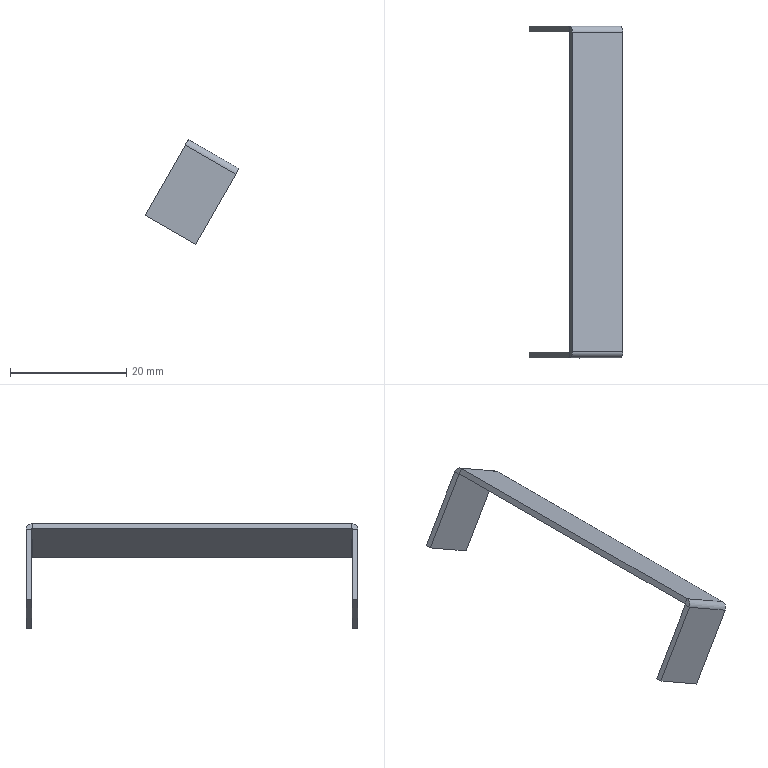Component | SolidWorks | FrontDoorFlangeWelding-2_WireRack-1 | 1 solid | 22 faces | box 16.13 x 57 x 17.99 mm | volume 845 mm3 | plane 18 | cylinder 4 | commonest cylinder face diameters 2.2 x2 0.2 x2
STEP:
#1=CARTESIAN_POINT('',(-0.3547,19.692,56.021));
#2=VERTEX_POINT('',#1);
#3=CARTESIAN_POINT('',(-0.01307,19.692,55.825));
#4=VERTEX_POINT('',#3);
#5=CARTESIAN_POINT('',(-0.3547,19.692,56.021));
#6=DIRECTION('',(0.8677,0.,-0.4971));
#7=VECTOR('',#6,39.37);
#8=LINE('',#5,#7);
#9=EDGE_CURVE('',#2,#4,#8,.T.);
#10=ORIENTED_EDGE('',*,*,#9,.F.);
#11=CARTESIAN_POINT('',(-0.3547,21.849,56.021));
#12=VERTEX_POINT('',#11);
#13=CARTESIAN_POINT('',(-0.3547,21.893,56.021));
#14=DIRECTION('',(0.,-1.,-0.));
#15=VECTOR('',#14,39.37);
#16=LINE('',#13,#15);
#17=EDGE_CURVE('',#12,#2,#16,.T.);
#18=ORIENTED_EDGE('',*,*,#17,.F.);
#19=CARTESIAN_POINT('',(-0.01307,21.849,55.825));
#20=VERTEX_POINT('',#19);
#21=CARTESIAN_POINT('',(-0.01307,21.849,55.825));
#22=DIRECTION('',(-0.8677,-0.,0.4971));
#23=VECTOR('',#22,39.37);
#24=LINE('',#21,#23);
#25=EDGE_CURVE('',#20,#12,#24,.T.);
#26=ORIENTED_EDGE('',*,*,#25,.F.);
#27=CARTESIAN_POINT('',(-0.01307,21.893,55.825));
#28=DIRECTION('',(-0.,1.,0.));
#29=VECTOR('',#28,39.37);
#30=LINE('',#27,#29);
#31=EDGE_CURVE('',#4,#20,#30,.T.);
#32=ORIENTED_EDGE('',*,*,#31,.F.);
#33=EDGE_LOOP('',(#10,#18,#26,#32));
#34=FACE_OUTER_BOUND('',#33,.T.);
#35=CARTESIAN_POINT('',(0.2035,19.647,55.701));
#36=DIRECTION('',(0.4971,-0.,0.8677));
#37=DIRECTION('',(0.8677,0.,-0.4971));
#38=AXIS2_PLACEMENT_3D('',#35,#36,#37);
#39=PLANE('',#38);
#40=ADVANCED_FACE('',(#34),#39,.F.);
#41=CARTESIAN_POINT('',(-0.3351,21.849,56.055));
#42=VERTEX_POINT('',#41);
#43=CARTESIAN_POINT('',(-0.3351,19.692,56.055));
#44=VERTEX_POINT('',#43);
#45=CARTESIAN_POINT('',(-0.3351,21.893,56.055));
#46=DIRECTION('',(0.,-1.,-0.));
#47=VECTOR('',#46,39.37);
#48=LINE('',#45,#47);
#49=EDGE_CURVE('',#42,#44,#48,.T.);
#50=ORIENTED_EDGE('',*,*,#49,.T.);
#51=CARTESIAN_POINT('',(0.006502,19.692,55.859));
#52=VERTEX_POINT('',#51);
#53=CARTESIAN_POINT('',(-0.3351,19.692,56.055));
#54=DIRECTION('',(0.8677,0.,-0.4971));
#55=VECTOR('',#54,39.37);
#56=LINE('',#53,#55);
#57=EDGE_CURVE('',#44,#52,#56,.T.);
#58=ORIENTED_EDGE('',*,*,#57,.T.);
#59=CARTESIAN_POINT('',(0.006502,21.849,55.859));
#60=VERTEX_POINT('',#59);
#61=CARTESIAN_POINT('',(0.006502,21.893,55.859));
#62=DIRECTION('',(-0.,1.,0.));
#63=VECTOR('',#62,39.37);
#64=LINE('',#61,#63);
#65=EDGE_CURVE('',#52,#60,#64,.T.);
#66=ORIENTED_EDGE('',*,*,#65,.T.);
#67=CARTESIAN_POINT('',(0.006502,21.849,55.859));
#68=DIRECTION('',(-0.8677,-0.,0.4971));
#69=VECTOR('',#68,39.37);
#70=LINE('',#67,#69);
#71=EDGE_CURVE('',#60,#42,#70,.T.);
#72=ORIENTED_EDGE('',*,*,#71,.T.);
#73=EDGE_LOOP('',(#50,#58,#66,#72));
#74=FACE_OUTER_BOUND('',#73,.T.);
#75=CARTESIAN_POINT('',(0.2231,19.647,55.735));
#76=DIRECTION('',(0.4971,-0.,0.8677));
#77=DIRECTION('',(0.8677,0.,-0.4971));
#78=AXIS2_PLACEMENT_3D('',#75,#76,#77);
#79=PLANE('',#78);
#80=ADVANCED_FACE('',(#74),#79,.T.);
#81=ORIENTED_EDGE('',*,*,#17,.T.);
#82=CARTESIAN_POINT('',(-0.3547,19.692,56.021));
#83=DIRECTION('',(0.4971,-0.,0.8677));
#84=VECTOR('',#83,39.37);
#85=LINE('',#82,#84);
#86=EDGE_CURVE('',#2,#44,#85,.T.);
#87=ORIENTED_EDGE('',*,*,#86,.T.);
#88=ORIENTED_EDGE('',*,*,#49,.F.);
#89=CARTESIAN_POINT('',(-0.3547,21.849,56.021));
#90=DIRECTION('',(0.4971,-0.,0.8677));
#91=VECTOR('',#90,39.37);
#92=LINE('',#89,#91);
#93=EDGE_CURVE('',#12,#42,#92,.T.);
#94=ORIENTED_EDGE('',*,*,#93,.F.);
#95=EDGE_LOOP('',(#81,#87,#88,#94));
#96=FACE_OUTER_BOUND('',#95,.T.);
#97=CARTESIAN_POINT('',(-0.3547,21.893,56.021));
#98=DIRECTION('',(-0.8677,-0.,0.4971));
#99=DIRECTION('',(0.4971,-0.,0.8677));
#100=AXIS2_PLACEMENT_3D('',#97,#98,#99);
#101=PLANE('',#100);
#102=ADVANCED_FACE('',(#96),#101,.T.);
#103=CARTESIAN_POINT('',(-0.01307,19.692,55.825));
#104=DIRECTION('',(0.4971,-0.,0.8677));
#105=VECTOR('',#104,39.37);
#106=LINE('',#103,#105);
#107=EDGE_CURVE('',#4,#52,#106,.T.);
#108=ORIENTED_EDGE('',*,*,#107,.F.);
#109=ORIENTED_EDGE('',*,*,#31,.T.);
#110=CARTESIAN_POINT('',(-0.01307,21.849,55.825));
#111=DIRECTION('',(0.4971,-0.,0.8677));
#112=VECTOR('',#111,39.37);
#113=LINE('',#110,#112);
#114=EDGE_CURVE('',#20,#60,#113,.T.);
#115=ORIENTED_EDGE('',*,*,#114,.T.);
#116=ORIENTED_EDGE('',*,*,#65,.F.);
#117=EDGE_LOOP('',(#108,#109,#115,#116));
#118=FACE_OUTER_BOUND('',#117,.T.);
#119=CARTESIAN_POINT('',(-0.01307,21.893,55.825));
#120=DIRECTION('',(0.8677,0.,-0.4971));
#121=DIRECTION('',(-0.,1.,0.));
#122=AXIS2_PLACEMENT_3D('',#119,#120,#121);
#123=PLANE('',#122);
#124=ADVANCED_FACE('',(#118),#123,.T.);
#125=CARTESIAN_POINT('',(-0.3566,21.853,56.017));
#126=VERTEX_POINT('',#125);
#127=CARTESIAN_POINT('',(-0.3566,21.893,56.017));
#128=VERTEX_POINT('',#127);
#129=CARTESIAN_POINT('',(-0.3566,21.893,56.017));
#130=DIRECTION('',(0.,1.,0.));
#131=VECTOR('',#130,39.37);
#132=LINE('',#129,#131);
#133=EDGE_CURVE('',#126,#128,#132,.T.);
#134=ORIENTED_EDGE('',*,*,#133,.F.);
#135=CARTESIAN_POINT('',(-0.3566,21.849,56.017));
#136=DIRECTION('',(-0.8677,-0.,0.4971));
#137=DIRECTION('',(-0.4971,0.,-0.8677));
#138=AXIS2_PLACEMENT_3D('',#135,#136,#137);
#139=CIRCLE('',#138,0.003937);
#140=EDGE_CURVE('',#12,#126,#139,.T.);
#141=ORIENTED_EDGE('',*,*,#140,.F.);
#142=ORIENTED_EDGE('',*,*,#93,.T.);
#143=CARTESIAN_POINT('',(-0.3566,21.849,56.017));
#144=DIRECTION('',(-0.8677,-0.,0.4971));
#145=DIRECTION('',(-0.4971,0.,-0.8677));
#146=AXIS2_PLACEMENT_3D('',#143,#144,#145);
#147=CIRCLE('',#146,0.04331);
#148=EDGE_CURVE('',#42,#128,#147,.T.);
#149=ORIENTED_EDGE('',*,*,#148,.T.);
#150=EDGE_LOOP('',(#134,#141,#142,#149));
#151=FACE_OUTER_BOUND('',#150,.T.);
#152=CARTESIAN_POINT('',(-0.3566,21.849,56.017));
#153=DIRECTION('',(-0.8677,-0.,0.4971));
#154=DIRECTION('',(0.4971,-0.,0.8677));
#155=AXIS2_PLACEMENT_3D('',#152,#153,#154);
#156=PLANE('',#155);
#157=ADVANCED_FACE('',(#151),#156,.T.);
#158=CARTESIAN_POINT('',(-0.01503,21.853,55.821));
#159=VERTEX_POINT('',#158);
#160=CARTESIAN_POINT('',(-0.01503,21.849,55.821));
#161=DIRECTION('',(0.8677,0.,-0.4971));
#162=DIRECTION('',(-0.4971,0.,-0.8677));
#163=AXIS2_PLACEMENT_3D('',#160,#161,#162);
#164=CIRCLE('',#163,0.003937);
#165=EDGE_CURVE('',#159,#20,#164,.T.);
#166=ORIENTED_EDGE('',*,*,#165,.F.);
#167=CARTESIAN_POINT('',(-0.01503,21.893,55.821));
#168=VERTEX_POINT('',#167);
#169=CARTESIAN_POINT('',(-0.01503,21.853,55.821));
#170=DIRECTION('',(0.,1.,0.));
#171=VECTOR('',#170,39.37);
#172=LINE('',#169,#171);
#173=EDGE_CURVE('',#159,#168,#172,.T.);
#174=ORIENTED_EDGE('',*,*,#173,.T.);
#175=CARTESIAN_POINT('',(-0.01503,21.849,55.821));
#176=DIRECTION('',(0.8677,0.,-0.4971));
#177=DIRECTION('',(-0.4971,0.,-0.8677));
#178=AXIS2_PLACEMENT_3D('',#175,#176,#177);
#179=CIRCLE('',#178,0.04331);
#180=EDGE_CURVE('',#168,#60,#179,.T.);
#181=ORIENTED_EDGE('',*,*,#180,.T.);
#182=ORIENTED_EDGE('',*,*,#114,.F.);
#183=EDGE_LOOP('',(#166,#174,#181,#182));
#184=FACE_OUTER_BOUND('',#183,.T.);
#185=CARTESIAN_POINT('',(-0.01503,21.849,55.821));
#186=DIRECTION('',(-0.8677,-0.,0.4971));
#187=DIRECTION('',(0.4971,-0.,0.8677));
#188=AXIS2_PLACEMENT_3D('',#185,#186,#187);
#189=PLANE('',#188);
#190=ADVANCED_FACE('',(#184),#189,.F.);
#191=ORIENTED_EDGE('',*,*,#71,.F.);
#192=ORIENTED_EDGE('',*,*,#180,.F.);
#193=CARTESIAN_POINT('',(0.2016,21.893,55.697));
#194=DIRECTION('',(0.8677,0.,-0.4971));
#195=VECTOR('',#194,39.37);
#196=LINE('',#193,#195);
#197=EDGE_CURVE('',#128,#168,#196,.T.);
#198=ORIENTED_EDGE('',*,*,#197,.F.);
#199=ORIENTED_EDGE('',*,*,#148,.F.);
#200=EDGE_LOOP('',(#191,#192,#198,#199));
#201=FACE_OUTER_BOUND('',#200,.T.);
#202=CARTESIAN_POINT('',(-0.01503,21.849,55.821));
#203=DIRECTION('',(0.8677,0.,-0.4971));
#204=DIRECTION('',(0.,1.,0.));
#205=AXIS2_PLACEMENT_3D('',#202,#203,#204);
#206=CYLINDRICAL_SURFACE('',#205,0.04331);
#207=ADVANCED_FACE('',(#201),#206,.T.);
#208=ORIENTED_EDGE('',*,*,#25,.T.);
#209=ORIENTED_EDGE('',*,*,#140,.T.);
#210=CARTESIAN_POINT('',(-0.3566,21.853,56.017));
#211=DIRECTION('',(0.8677,0.,-0.4971));
#212=VECTOR('',#211,39.37);
#213=LINE('',#210,#212);
#214=EDGE_CURVE('',#126,#159,#213,.T.);
#215=ORIENTED_EDGE('',*,*,#214,.T.);
#216=ORIENTED_EDGE('',*,*,#165,.T.);
#217=EDGE_LOOP('',(#208,#209,#215,#216));
#218=FACE_OUTER_BOUND('',#217,.T.);
#219=CARTESIAN_POINT('',(-0.01503,21.849,55.821));
#220=DIRECTION('',(0.8677,0.,-0.4971));
#221=DIRECTION('',(0.,1.,0.));
#222=AXIS2_PLACEMENT_3D('',#219,#220,#221);
#223=CYLINDRICAL_SURFACE('',#222,0.003937);
#224=ADVANCED_FACE('',(#218),#223,.F.);
#225=CARTESIAN_POINT('',(-0.2871,21.893,55.347));
#226=VERTEX_POINT('',#225);
#227=CARTESIAN_POINT('',(-0.01307,21.893,55.825));
#228=DIRECTION('',(0.4971,-0.,0.8677));
#229=VECTOR('',#228,39.37);
#230=LINE('',#227,#229);
#231=EDGE_CURVE('',#226,#168,#230,.T.);
#232=ORIENTED_EDGE('',*,*,#231,.T.);
#233=ORIENTED_EDGE('',*,*,#173,.F.);
#234=CARTESIAN_POINT('',(-0.2871,21.853,55.347));
#235=VERTEX_POINT('',#234);
#236=CARTESIAN_POINT('',(0.006502,21.853,55.859));
#237=DIRECTION('',(0.4971,-0.,0.8677));
#238=VECTOR('',#237,39.37);
#239=LINE('',#236,#238);
#240=EDGE_CURVE('',#235,#159,#239,.T.);
#241=ORIENTED_EDGE('',*,*,#240,.F.);
#242=CARTESIAN_POINT('',(-0.2871,21.893,55.347));
#243=DIRECTION('',(-0.,-1.,-0.));
#244=VECTOR('',#243,39.37);
#245=LINE('',#242,#244);
#246=EDGE_CURVE('',#226,#235,#245,.T.);
#247=ORIENTED_EDGE('',*,*,#246,.F.);
#248=EDGE_LOOP('',(#232,#233,#241,#247));
#249=FACE_OUTER_BOUND('',#248,.T.);
#250=CARTESIAN_POINT('',(-0.01307,21.893,55.825));
#251=DIRECTION('',(0.8677,0.,-0.4971));
#252=DIRECTION('',(-0.4971,0.,-0.8677));
#253=AXIS2_PLACEMENT_3D('',#250,#251,#252);
#254=PLANE('',#253);
#255=ADVANCED_FACE('',(#249),#254,.T.);
#256=CARTESIAN_POINT('',(-0.6287,21.853,55.542));
#257=VERTEX_POINT('',#256);
#258=CARTESIAN_POINT('',(-0.3351,21.853,56.055));
#259=DIRECTION('',(-0.4971,0.,-0.8677));
#260=VECTOR('',#259,39.37);
#261=LINE('',#258,#260);
#262=EDGE_CURVE('',#126,#257,#261,.T.);
#263=ORIENTED_EDGE('',*,*,#262,.F.);
#264=ORIENTED_EDGE('',*,*,#133,.T.);
#265=CARTESIAN_POINT('',(-0.6287,21.893,55.542));
#266=VERTEX_POINT('',#265);
#267=CARTESIAN_POINT('',(-0.6287,21.893,55.542));
#268=DIRECTION('',(-0.4971,0.,-0.8677));
#269=VECTOR('',#268,39.37);
#270=LINE('',#267,#269);
#271=EDGE_CURVE('',#128,#266,#270,.T.);
#272=ORIENTED_EDGE('',*,*,#271,.T.);
#273=CARTESIAN_POINT('',(-0.6287,21.893,55.542));
#274=DIRECTION('',(-0.,-1.,-0.));
#275=VECTOR('',#274,39.37);
#276=LINE('',#273,#275);
#277=EDGE_CURVE('',#266,#257,#276,.T.);
#278=ORIENTED_EDGE('',*,*,#277,.T.);
#279=EDGE_LOOP('',(#263,#264,#272,#278));
#280=FACE_OUTER_BOUND('',#279,.T.);
#281=CARTESIAN_POINT('',(-0.6287,21.893,55.542));
#282=DIRECTION('',(-0.8677,-0.,0.4971));
#283=DIRECTION('',(0.4971,-0.,0.8677));
#284=AXIS2_PLACEMENT_3D('',#281,#282,#283);
#285=PLANE('',#284);
#286=ADVANCED_FACE('',(#280),#285,.T.);
#287=ORIENTED_EDGE('',*,*,#271,.F.);
#288=ORIENTED_EDGE('',*,*,#197,.T.);
#289=ORIENTED_EDGE('',*,*,#231,.F.);
#290=CARTESIAN_POINT('',(-0.2871,21.893,55.347));
#291=DIRECTION('',(0.8677,0.,-0.4971));
#292=VECTOR('',#291,39.37);
#293=LINE('',#290,#292);
#294=EDGE_CURVE('',#266,#226,#293,.T.);
#295=ORIENTED_EDGE('',*,*,#294,.F.);
#296=EDGE_LOOP('',(#287,#288,#289,#295));
#297=FACE_OUTER_BOUND('',#296,.T.);
#298=CARTESIAN_POINT('',(0.2231,21.893,55.735));
#299=DIRECTION('',(0.,1.,0.));
#300=DIRECTION('',(0.4971,-0.,0.8677));
#301=AXIS2_PLACEMENT_3D('',#298,#299,#300);
#302=PLANE('',#301);
#303=ADVANCED_FACE('',(#297),#302,.T.);
#304=ORIENTED_EDGE('',*,*,#214,.F.);
#305=ORIENTED_EDGE('',*,*,#262,.T.);
#306=CARTESIAN_POINT('',(-0.07047,21.853,55.223));
#307=DIRECTION('',(0.8677,0.,-0.4971));
#308=VECTOR('',#307,39.37);
#309=LINE('',#306,#308);
#310=EDGE_CURVE('',#257,#235,#309,.T.);
#311=ORIENTED_EDGE('',*,*,#310,.T.);
#312=ORIENTED_EDGE('',*,*,#240,.T.);
#313=EDGE_LOOP('',(#304,#305,#311,#312));
#314=FACE_OUTER_BOUND('',#313,.T.);
#315=CARTESIAN_POINT('',(0.2231,21.853,55.735));
#316=DIRECTION('',(0.,1.,0.));
#317=DIRECTION('',(0.4971,-0.,0.8677));
#318=AXIS2_PLACEMENT_3D('',#315,#316,#317);
#319=PLANE('',#318);
#320=ADVANCED_FACE('',(#314),#319,.F.);
#321=ORIENTED_EDGE('',*,*,#310,.F.);
#322=ORIENTED_EDGE('',*,*,#277,.F.);
#323=ORIENTED_EDGE('',*,*,#294,.T.);
#324=ORIENTED_EDGE('',*,*,#246,.T.);
#325=EDGE_LOOP('',(#321,#322,#323,#324));
#326=FACE_OUTER_BOUND('',#325,.T.);
#327=CARTESIAN_POINT('',(-0.2871,21.893,55.347));
#328=DIRECTION('',(-0.4971,0.,-0.8677));
#329=DIRECTION('',(0.,1.,0.));
#330=AXIS2_PLACEMENT_3D('',#327,#328,#329);
#331=PLANE('',#330);
#332=ADVANCED_FACE('',(#326),#331,.T.);
#333=CARTESIAN_POINT('',(-0.01503,19.688,55.821));
#334=VERTEX_POINT('',#333);
#335=CARTESIAN_POINT('',(-0.01503,19.649,55.821));
#336=VERTEX_POINT('',#335);
#337=CARTESIAN_POINT('',(-0.01503,19.649,55.821));
#338=DIRECTION('',(0.,-1.,-0.));
#339=VECTOR('',#338,39.37);
#340=LINE('',#337,#339);
#341=EDGE_CURVE('',#334,#336,#340,.T.);
#342=ORIENTED_EDGE('',*,*,#341,.F.);
#343=CARTESIAN_POINT('',(-0.01503,19.692,55.821));
#344=DIRECTION('',(0.8677,0.,-0.4971));
#345=DIRECTION('',(0.4971,0.,0.8677));
#346=AXIS2_PLACEMENT_3D('',#343,#344,#345);
#347=CIRCLE('',#346,0.003937);
#348=EDGE_CURVE('',#4,#334,#347,.T.);
#349=ORIENTED_EDGE('',*,*,#348,.F.);
#350=ORIENTED_EDGE('',*,*,#107,.T.);
#351=CARTESIAN_POINT('',(-0.01503,19.692,55.821));
#352=DIRECTION('',(0.8677,0.,-0.4971));
#353=DIRECTION('',(0.4971,0.,0.8677));
#354=AXIS2_PLACEMENT_3D('',#351,#352,#353);
#355=CIRCLE('',#354,0.04331);
#356=EDGE_CURVE('',#52,#336,#355,.T.);
#357=ORIENTED_EDGE('',*,*,#356,.T.);
#358=EDGE_LOOP('',(#342,#349,#350,#357));
#359=FACE_OUTER_BOUND('',#358,.T.);
#360=CARTESIAN_POINT('',(-0.01503,19.692,55.821));
#361=DIRECTION('',(0.8677,0.,-0.4971));
#362=DIRECTION('',(-0.4971,0.,-0.8677));
#363=AXIS2_PLACEMENT_3D('',#360,#361,#362);
#364=PLANE('',#363);
#365=ADVANCED_FACE('',(#359),#364,.T.);
#366=CARTESIAN_POINT('',(-0.3566,19.688,56.017));
#367=VERTEX_POINT('',#366);
#368=CARTESIAN_POINT('',(-0.3566,19.692,56.017));
#369=DIRECTION('',(-0.8677,-0.,0.4971));
#370=DIRECTION('',(0.4971,0.,0.8677));
#371=AXIS2_PLACEMENT_3D('',#368,#369,#370);
#372=CIRCLE('',#371,0.003937);
#373=EDGE_CURVE('',#367,#2,#372,.T.);
#374=ORIENTED_EDGE('',*,*,#373,.F.);
#375=CARTESIAN_POINT('',(-0.3566,19.649,56.017));
#376=VERTEX_POINT('',#375);
#377=CARTESIAN_POINT('',(-0.3566,19.688,56.017));
#378=DIRECTION('',(0.,-1.,-0.));
#379=VECTOR('',#378,39.37);
#380=LINE('',#377,#379);
#381=EDGE_CURVE('',#367,#376,#380,.T.);
#382=ORIENTED_EDGE('',*,*,#381,.T.);
#383=CARTESIAN_POINT('',(-0.3566,19.692,56.017));
#384=DIRECTION('',(-0.8677,-0.,0.4971));
#385=DIRECTION('',(0.4971,0.,0.8677));
#386=AXIS2_PLACEMENT_3D('',#383,#384,#385);
#387=CIRCLE('',#386,0.04331);
#388=EDGE_CURVE('',#376,#44,#387,.T.);
#389=ORIENTED_EDGE('',*,*,#388,.T.);
#390=ORIENTED_EDGE('',*,*,#86,.F.);
#391=EDGE_LOOP('',(#374,#382,#389,#390));
#392=FACE_OUTER_BOUND('',#391,.T.);
#393=CARTESIAN_POINT('',(-0.3566,19.692,56.017));
#394=DIRECTION('',(0.8677,0.,-0.4971));
#395=DIRECTION('',(-0.4971,0.,-0.8677));
#396=AXIS2_PLACEMENT_3D('',#393,#394,#395);
#397=PLANE('',#396);
#398=ADVANCED_FACE('',(#392),#397,.F.);
#399=ORIENTED_EDGE('',*,*,#57,.F.);
#400=ORIENTED_EDGE('',*,*,#388,.F.);
#401=CARTESIAN_POINT('',(0.2016,19.649,55.697));
#402=DIRECTION('',(-0.8677,-0.,0.4971));
#403=VECTOR('',#402,39.37);
#404=LINE('',#401,#403);
#405=EDGE_CURVE('',#336,#376,#404,.T.);
#406=ORIENTED_EDGE('',*,*,#405,.F.);
#407=ORIENTED_EDGE('',*,*,#356,.F.);
#408=EDGE_LOOP('',(#399,#400,#406,#407));
#409=FACE_OUTER_BOUND('',#408,.T.);
#410=CARTESIAN_POINT('',(-0.3566,19.692,56.017));
#411=DIRECTION('',(-0.8677,-0.,0.4971));
#412=DIRECTION('',(0.,-1.,0.));
#413=AXIS2_PLACEMENT_3D('',#410,#411,#412);
#414=CYLINDRICAL_SURFACE('',#413,0.04331);
#415=ADVANCED_FACE('',(#409),#414,.T.);
#416=ORIENTED_EDGE('',*,*,#9,.T.);
#417=ORIENTED_EDGE('',*,*,#348,.T.);
#418=CARTESIAN_POINT('',(-0.01503,19.688,55.821));
#419=DIRECTION('',(-0.8677,-0.,0.4971));
#420=VECTOR('',#419,39.37);
#421=LINE('',#418,#420);
#422=EDGE_CURVE('',#334,#367,#421,.T.);
#423=ORIENTED_EDGE('',*,*,#422,.T.);
#424=ORIENTED_EDGE('',*,*,#373,.T.);
#425=EDGE_LOOP('',(#416,#417,#423,#424));
#426=FACE_OUTER_BOUND('',#425,.T.);
#427=CARTESIAN_POINT('',(-0.3566,19.692,56.017));
#428=DIRECTION('',(-0.8677,-0.,0.4971));
#429=DIRECTION('',(0.,-1.,0.));
#430=AXIS2_PLACEMENT_3D('',#427,#428,#429);
#431=CYLINDRICAL_SURFACE('',#430,0.003937);
#432=ADVANCED_FACE('',(#426),#431,.F.);
#433=CARTESIAN_POINT('',(-0.6287,19.649,55.542));
#434=VERTEX_POINT('',#433);
#435=CARTESIAN_POINT('',(-0.3547,19.649,56.021));
#436=DIRECTION('',(0.4971,-0.,0.8677));
#437=VECTOR('',#436,39.37);
#438=LINE('',#435,#437);
#439=EDGE_CURVE('',#434,#376,#438,.T.);
#440=ORIENTED_EDGE('',*,*,#439,.T.);
#441=ORIENTED_EDGE('',*,*,#381,.F.);
#442=CARTESIAN_POINT('',(-0.6287,19.688,55.542));
#443=VERTEX_POINT('',#442);
#444=CARTESIAN_POINT('',(-0.3351,19.688,56.055));
#445=DIRECTION('',(0.4971,-0.,0.8677));
#446=VECTOR('',#445,39.37);
#447=LINE('',#444,#446);
#448=EDGE_CURVE('',#443,#367,#447,.T.);
#449=ORIENTED_EDGE('',*,*,#448,.F.);
#450=CARTESIAN_POINT('',(-0.6287,19.649,55.542));
#451=DIRECTION('',(-0.,1.,0.));
#452=VECTOR('',#451,39.37);
#453=LINE('',#450,#452);
#454=EDGE_CURVE('',#434,#443,#453,.T.);
#455=ORIENTED_EDGE('',*,*,#454,.F.);
#456=EDGE_LOOP('',(#440,#441,#449,#455));
#457=FACE_OUTER_BOUND('',#456,.T.);
#458=CARTESIAN_POINT('',(-0.3547,19.649,56.021));
#459=DIRECTION('',(-0.8677,-0.,0.4971));
#460=DIRECTION('',(0.4971,-0.,0.8677));
#461=AXIS2_PLACEMENT_3D('',#458,#459,#460);
#462=PLANE('',#461);
#463=ADVANCED_FACE('',(#457),#462,.T.);
#464=CARTESIAN_POINT('',(-0.2871,19.688,55.347));
#465=VERTEX_POINT('',#464);
#466=CARTESIAN_POINT('',(0.006502,19.688,55.859));
#467=DIRECTION('',(-0.4971,0.,-0.8677));
#468=VECTOR('',#467,39.37);
#469=LINE('',#466,#468);
#470=EDGE_CURVE('',#334,#465,#469,.T.);
#471=ORIENTED_EDGE('',*,*,#470,.F.);
#472=ORIENTED_EDGE('',*,*,#341,.T.);
#473=CARTESIAN_POINT('',(-0.2871,19.649,55.347));
#474=VERTEX_POINT('',#473);
#475=CARTESIAN_POINT('',(-0.2871,19.649,55.347));
#476=DIRECTION('',(-0.4971,0.,-0.8677));
#477=VECTOR('',#476,39.37);
#478=LINE('',#475,#477);
#479=EDGE_CURVE('',#336,#474,#478,.T.);
#480=ORIENTED_EDGE('',*,*,#479,.T.);
#481=CARTESIAN_POINT('',(-0.2871,19.649,55.347));
#482=DIRECTION('',(-0.,1.,0.));
#483=VECTOR('',#482,39.37);
#484=LINE('',#481,#483);
#485=EDGE_CURVE('',#474,#465,#484,.T.);
#486=ORIENTED_EDGE('',*,*,#485,.T.);
#487=EDGE_LOOP('',(#471,#472,#480,#486));
#488=FACE_OUTER_BOUND('',#487,.T.);
#489=CARTESIAN_POINT('',(-0.2871,19.649,55.347));
#490=DIRECTION('',(0.8677,0.,-0.4971));
#491=DIRECTION('',(-0.4971,0.,-0.8677));
#492=AXIS2_PLACEMENT_3D('',#489,#490,#491);
#493=PLANE('',#492);
#494=ADVANCED_FACE('',(#488),#493,.T.);
#495=ORIENTED_EDGE('',*,*,#479,.F.);
#496=ORIENTED_EDGE('',*,*,#405,.T.);
#497=ORIENTED_EDGE('',*,*,#439,.F.);
#498=CARTESIAN_POINT('',(-0.6287,19.649,55.542));
#499=DIRECTION('',(-0.8677,-0.,0.4971));
#500=VECTOR('',#499,39.37);
#501=LINE('',#498,#500);
#502=EDGE_CURVE('',#474,#434,#501,.T.);
#503=ORIENTED_EDGE('',*,*,#502,.F.);
#504=EDGE_LOOP('',(#495,#496,#497,#503));
#505=FACE_OUTER_BOUND('',#504,.T.);
#506=CARTESIAN_POINT('',(0.2231,19.649,55.735));
#507=DIRECTION('',(0.,-1.,-0.));
#508=DIRECTION('',(-0.4971,0.,-0.8677));
#509=AXIS2_PLACEMENT_3D('',#506,#507,#508);
#510=PLANE('',#509);
#511=ADVANCED_FACE('',(#505),#510,.T.);
#512=ORIENTED_EDGE('',*,*,#422,.F.);
#513=ORIENTED_EDGE('',*,*,#470,.T.);
#514=CARTESIAN_POINT('',(-0.07047,19.688,55.223));
#515=DIRECTION('',(-0.8677,-0.,0.4971));
#516=VECTOR('',#515,39.37);
#517=LINE('',#514,#516);
#518=EDGE_CURVE('',#465,#443,#517,.T.);
#519=ORIENTED_EDGE('',*,*,#518,.T.);
#520=ORIENTED_EDGE('',*,*,#448,.T.);
#521=EDGE_LOOP('',(#512,#513,#519,#520));
#522=FACE_OUTER_BOUND('',#521,.T.);
#523=CARTESIAN_POINT('',(0.2231,19.688,55.735));
#524=DIRECTION('',(0.,-1.,-0.));
#525=DIRECTION('',(-0.4971,0.,-0.8677));
#526=AXIS2_PLACEMENT_3D('',#523,#524,#525);
#527=PLANE('',#526);
#528=ADVANCED_FACE('',(#522),#527,.F.);
#529=ORIENTED_EDGE('',*,*,#518,.F.);
#530=ORIENTED_EDGE('',*,*,#485,.F.);
#531=ORIENTED_EDGE('',*,*,#502,.T.);
#532=ORIENTED_EDGE('',*,*,#454,.T.);
#533=EDGE_LOOP('',(#529,#530,#531,#532));
#534=FACE_OUTER_BOUND('',#533,.T.);
#535=CARTESIAN_POINT('',(-0.6287,19.649,55.542));
#536=DIRECTION('',(-0.4971,0.,-0.8677));
#537=DIRECTION('',(-0.,1.,0.));
#538=AXIS2_PLACEMENT_3D('',#535,#536,#537);
#539=PLANE('',#538);
#540=ADVANCED_FACE('',(#534),#539,.T.);
#541=CLOSED_SHELL('',(#40,#80,#102,#124,#157,#190,#207,#224,#255,#286,#303,#320,#332,#365,#398,#415,#432,#463,#494,#511,#528,#540));
#542=MANIFOLD_SOLID_BREP('',#541);
#543=CARTESIAN_POINT('',(0.,0.,0.));
#544=DIRECTION('',(0.,0.,1.));
#545=DIRECTION('',(1.,0.,0.));
#546=AXIS2_PLACEMENT_3D('',#543,#544,#545);
#547=(LENGTH_UNIT()NAMED_UNIT(*)SI_UNIT($,.METRE.));
#548=LENGTH_MEASURE_WITH_UNIT(LENGTH_MEASURE(0.0254),#547);
#549=DIMENSIONAL_EXPONENTS(1.,0.,0.,0.,0.,0.,0.);
#550=(CONVERSION_BASED_UNIT('',#548)LENGTH_UNIT()NAMED_UNIT(#549));
#551=UNCERTAINTY_MEASURE_WITH_UNIT(LENGTH_MEASURE(0.00001),#550,'','');
#552=(NAMED_UNIT(*)PLANE_ANGLE_UNIT()SI_UNIT($,.RADIAN.));
#553=(NAMED_UNIT(*)SI_UNIT($,.STERADIAN.)SOLID_ANGLE_UNIT());
#554=(GEOMETRIC_REPRESENTATION_CONTEXT(3)GLOBAL_UNCERTAINTY_ASSIGNED_CONTEXT((#551))GLOBAL_UNIT_ASSIGNED_CONTEXT((#550,#552,#553))REPRESENTATION_CONTEXT('',''));
#555=ADVANCED_BREP_SHAPE_REPRESENTATION('',(#542,#546),#554);
#556=COLOUR_RGB('',0.7922,0.8196,0.9333);
#557=FILL_AREA_STYLE_COLOUR('',#556);
#558=FILL_AREA_STYLE('',(#557));
#559=SURFACE_STYLE_FILL_AREA(#558);
#560=SURFACE_SIDE_STYLE('',(#559));
#561=SURFACE_STYLE_USAGE(.BOTH.,#560);
#562=PRESENTATION_STYLE_ASSIGNMENT((#561));
#563=STYLED_ITEM('',(#562),#542);
#564=(LENGTH_UNIT()NAMED_UNIT(*)SI_UNIT($,.METRE.));
#565=LENGTH_MEASURE_WITH_UNIT(LENGTH_MEASURE(0.0254),#564);
#566=DIMENSIONAL_EXPONENTS(1.,0.,0.,0.,0.,0.,0.);
#567=(CONVERSION_BASED_UNIT('',#565)LENGTH_UNIT()NAMED_UNIT(#566));
#568=UNCERTAINTY_MEASURE_WITH_UNIT(LENGTH_MEASURE(0.00001),#567,'','');
#569=(NAMED_UNIT(*)PLANE_ANGLE_UNIT()SI_UNIT($,.RADIAN.));
#570=(NAMED_UNIT(*)SI_UNIT($,.STERADIAN.)SOLID_ANGLE_UNIT());
#571=(GEOMETRIC_REPRESENTATION_CONTEXT(3)GLOBAL_UNCERTAINTY_ASSIGNED_CONTEXT((#568))GLOBAL_UNIT_ASSIGNED_CONTEXT((#567,#569,#570))REPRESENTATION_CONTEXT('',''));
#572=MECHANICAL_DESIGN_GEOMETRIC_PRESENTATION_REPRESENTATION('',(#563),#571);
#573=PRESENTATION_LAYER_ASSIGNMENT('','',(#563));